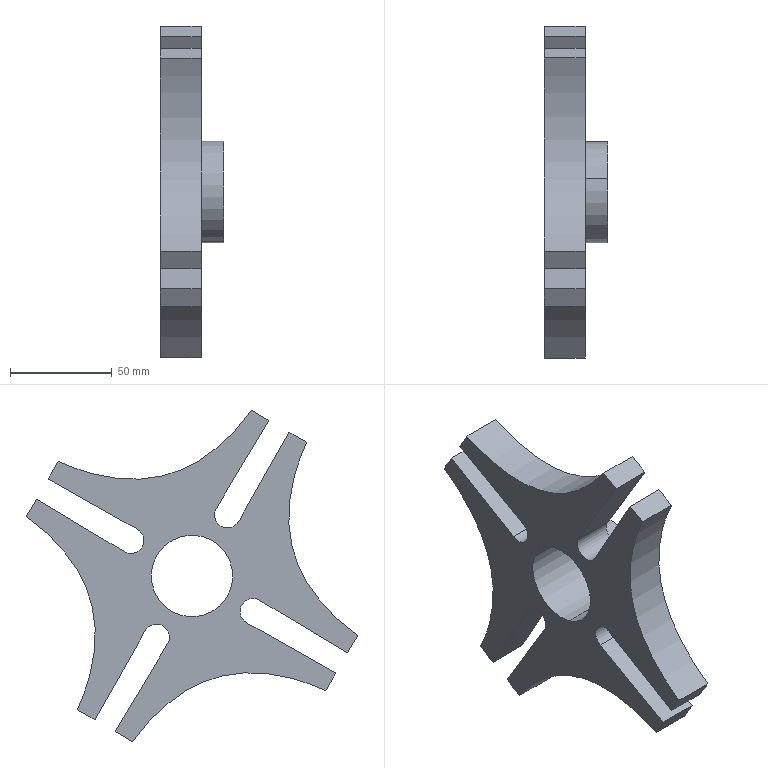Component | SolidWorks | GrooveWheel-2 | 1 solid | 33 faces | box 31 x 162.73 x 162.73 mm | volume 210042 mm3 | plane 19 | cylinder 10 | spline 4 | commonest cylinder face diameters 12.728 x6 40 x2 50 x2
STEP:
#1=CARTESIAN_POINT('',(15.611,0.8047,-8.688));
#2=VERTEX_POINT('',#1);
#3=CARTESIAN_POINT('',(15.611,0.4008,-10.21));
#4=VERTEX_POINT('',#3);
#5=CARTESIAN_POINT('',(15.611,0.6028,-9.449));
#6=DIRECTION('',(1.,0.,0.));
#7=DIRECTION('',(0.,-0.2564,-0.9666));
#8=AXIS2_PLACEMENT_3D('',#5,#6,#7);
#9=CIRCLE('',#8,0.7874);
#10=EDGE_CURVE('',#2,#4,#9,.T.);
#11=ORIENTED_EDGE('',*,*,#10,.T.);
#12=CARTESIAN_POINT('',(14.391,0.4008,-10.21));
#13=VERTEX_POINT('',#12);
#14=CARTESIAN_POINT('',(15.611,0.4008,-10.21));
#15=DIRECTION('',(-1.,0.,0.));
#16=VECTOR('',#15,39.37);
#17=LINE('',#14,#16);
#18=EDGE_CURVE('',#4,#13,#17,.T.);
#19=ORIENTED_EDGE('',*,*,#18,.T.);
#20=CARTESIAN_POINT('',(14.391,0.8047,-8.688));
#21=VERTEX_POINT('',#20);
#22=CARTESIAN_POINT('',(14.391,0.6028,-9.449));
#23=DIRECTION('',(1.,0.,0.));
#24=DIRECTION('',(0.,-0.2564,-0.9666));
#25=AXIS2_PLACEMENT_3D('',#22,#23,#24);
#26=CIRCLE('',#25,0.7874);
#27=EDGE_CURVE('',#21,#13,#26,.T.);
#28=ORIENTED_EDGE('',*,*,#27,.F.);
#29=CARTESIAN_POINT('',(15.611,0.8047,-8.688));
#30=DIRECTION('',(-1.,0.,0.));
#31=VECTOR('',#30,39.37);
#32=LINE('',#29,#31);
#33=EDGE_CURVE('',#2,#21,#32,.T.);
#34=ORIENTED_EDGE('',*,*,#33,.F.);
#35=EDGE_LOOP('',(#11,#19,#28,#34));
#36=FACE_OUTER_BOUND('',#35,.T.);
#37=CARTESIAN_POINT('',(15.611,0.6028,-9.449));
#38=DIRECTION('',(-1.,0.,0.));
#39=DIRECTION('',(0.,0.2564,0.9666));
#40=AXIS2_PLACEMENT_3D('',#37,#38,#39);
#41=CYLINDRICAL_SURFACE('',#40,0.7874);
#42=ADVANCED_FACE('',(#36),#41,.F.);
#43=CARTESIAN_POINT('',(15.611,0.3504,-10.4));
#44=VERTEX_POINT('',#43);
#45=CARTESIAN_POINT('',(15.611,0.8552,-8.497));
#46=VERTEX_POINT('',#45);
#47=CARTESIAN_POINT('',(15.611,0.6028,-9.449));
#48=DIRECTION('',(1.,0.,0.));
#49=DIRECTION('',(0.,-0.2564,-0.9666));
#50=AXIS2_PLACEMENT_3D('',#47,#48,#49);
#51=CIRCLE('',#50,0.9843);
#52=EDGE_CURVE('',#44,#46,#51,.T.);
#53=ORIENTED_EDGE('',*,*,#52,.F.);
#54=CARTESIAN_POINT('',(15.178,0.3504,-10.4));
#55=VERTEX_POINT('',#54);
#56=CARTESIAN_POINT('',(15.611,0.3504,-10.4));
#57=DIRECTION('',(-1.,0.,0.));
#58=VECTOR('',#57,39.37);
#59=LINE('',#56,#58);
#60=EDGE_CURVE('',#44,#55,#59,.T.);
#61=ORIENTED_EDGE('',*,*,#60,.T.);
#62=CARTESIAN_POINT('',(15.178,0.8552,-8.497));
#63=VERTEX_POINT('',#62);
#64=CARTESIAN_POINT('',(15.178,0.6028,-9.449));
#65=DIRECTION('',(1.,0.,0.));
#66=DIRECTION('',(0.,-0.2564,-0.9666));
#67=AXIS2_PLACEMENT_3D('',#64,#65,#66);
#68=CIRCLE('',#67,0.9843);
#69=EDGE_CURVE('',#55,#63,#68,.T.);
#70=ORIENTED_EDGE('',*,*,#69,.T.);
#71=CARTESIAN_POINT('',(15.611,0.8552,-8.497));
#72=DIRECTION('',(-1.,0.,0.));
#73=VECTOR('',#72,39.37);
#74=LINE('',#71,#73);
#75=EDGE_CURVE('',#46,#63,#74,.T.);
#76=ORIENTED_EDGE('',*,*,#75,.F.);
#77=EDGE_LOOP('',(#53,#61,#70,#76));
#78=FACE_OUTER_BOUND('',#77,.T.);
#79=CARTESIAN_POINT('',(15.611,0.6028,-9.449));
#80=DIRECTION('',(-1.,0.,0.));
#81=DIRECTION('',(0.,0.2564,0.9666));
#82=AXIS2_PLACEMENT_3D('',#79,#80,#81);
#83=CYLINDRICAL_SURFACE('',#82,0.9843);
#84=ADVANCED_FACE('',(#78),#83,.T.);
#85=CARTESIAN_POINT('',(15.178,1.508,-10.509));
#86=VERTEX_POINT('',#85);
#87=CARTESIAN_POINT('',(15.178,1.352,-10.386));
#88=VERTEX_POINT('',#87);
#89=CARTESIAN_POINT('',(15.178,1.288,-10.628));
#90=DIRECTION('',(1.,0.,0.));
#91=DIRECTION('',(0.,-0.2564,-0.9666));
#92=AXIS2_PLACEMENT_3D('',#89,#90,#91);
#93=CIRCLE('',#92,0.2505);
#94=EDGE_CURVE('',#86,#88,#93,.T.);
#95=ORIENTED_EDGE('',*,*,#94,.T.);
#96=CARTESIAN_POINT('',(14.391,1.352,-10.386));
#97=VERTEX_POINT('',#96);
#98=CARTESIAN_POINT('',(15.178,1.352,-10.386));
#99=DIRECTION('',(-1.,0.,0.));
#100=VECTOR('',#99,39.37);
#101=LINE('',#98,#100);
#102=EDGE_CURVE('',#88,#97,#101,.T.);
#103=ORIENTED_EDGE('',*,*,#102,.T.);
#104=CARTESIAN_POINT('',(14.391,1.508,-10.509));
#105=VERTEX_POINT('',#104);
#106=CARTESIAN_POINT('',(14.391,1.288,-10.628));
#107=DIRECTION('',(1.,0.,0.));
#108=DIRECTION('',(0.,-0.2564,-0.9666));
#109=AXIS2_PLACEMENT_3D('',#106,#107,#108);
#110=CIRCLE('',#109,0.2505);
#111=EDGE_CURVE('',#105,#97,#110,.T.);
#112=ORIENTED_EDGE('',*,*,#111,.F.);
#113=CARTESIAN_POINT('',(15.178,1.508,-10.509));
#114=DIRECTION('',(-1.,0.,0.));
#115=VECTOR('',#114,39.37);
#116=LINE('',#113,#115);
#117=EDGE_CURVE('',#86,#105,#116,.T.);
#118=ORIENTED_EDGE('',*,*,#117,.F.);
#119=EDGE_LOOP('',(#95,#103,#112,#118));
#120=FACE_OUTER_BOUND('',#119,.T.);
#121=CARTESIAN_POINT('',(15.178,1.288,-10.628));
#122=DIRECTION('',(-1.,0.,0.));
#123=DIRECTION('',(0.,0.2564,0.9666));
#124=AXIS2_PLACEMENT_3D('',#121,#122,#123);
#125=CYLINDRICAL_SURFACE('',#124,0.2505);
#126=ADVANCED_FACE('',(#120),#125,.F.);
#127=CARTESIAN_POINT('',(15.178,-0.4572,-10.354));
#128=VERTEX_POINT('',#127);
#129=CARTESIAN_POINT('',(15.178,-0.5127,-9.892));
#130=VERTEX_POINT('',#129);
#131=CARTESIAN_POINT('',(15.178,-0.5769,-10.134));
#132=DIRECTION('',(1.,0.,0.));
#133=DIRECTION('',(0.,-0.2564,-0.9666));
#134=AXIS2_PLACEMENT_3D('',#131,#132,#133);
#135=CIRCLE('',#134,0.2505);
#136=EDGE_CURVE('',#128,#130,#135,.T.);
#137=ORIENTED_EDGE('',*,*,#136,.T.);
#138=CARTESIAN_POINT('',(14.391,-0.5127,-9.892));
#139=VERTEX_POINT('',#138);
#140=CARTESIAN_POINT('',(15.178,-0.5127,-9.892));
#141=DIRECTION('',(-1.,0.,0.));
#142=VECTOR('',#141,39.37);
#143=LINE('',#140,#142);
#144=EDGE_CURVE('',#130,#139,#143,.T.);
#145=ORIENTED_EDGE('',*,*,#144,.T.);
#146=CARTESIAN_POINT('',(14.391,-0.4572,-10.354));
#147=VERTEX_POINT('',#146);
#148=CARTESIAN_POINT('',(14.391,-0.5769,-10.134));
#149=DIRECTION('',(1.,0.,0.));
#150=DIRECTION('',(0.,-0.2564,-0.9666));
#151=AXIS2_PLACEMENT_3D('',#148,#149,#150);
#152=CIRCLE('',#151,0.2505);
#153=EDGE_CURVE('',#147,#139,#152,.T.);
#154=ORIENTED_EDGE('',*,*,#153,.F.);
#155=CARTESIAN_POINT('',(15.178,-0.4572,-10.354));
#156=DIRECTION('',(-1.,0.,0.));
#157=VECTOR('',#156,39.37);
#158=LINE('',#155,#157);
#159=EDGE_CURVE('',#128,#147,#158,.T.);
#160=ORIENTED_EDGE('',*,*,#159,.F.);
#161=EDGE_LOOP('',(#137,#145,#154,#160));
#162=FACE_OUTER_BOUND('',#161,.T.);
#163=CARTESIAN_POINT('',(15.178,-0.5769,-10.134));
#164=DIRECTION('',(-1.,0.,0.));
#165=DIRECTION('',(0.,0.2564,0.9666));
#166=AXIS2_PLACEMENT_3D('',#163,#164,#165);
#167=CYLINDRICAL_SURFACE('',#166,0.2505);
#168=ADVANCED_FACE('',(#162),#167,.F.);
#169=CARTESIAN_POINT('',(15.178,-0.5444,-6.246));
#170=VERTEX_POINT('',#169);
#171=CARTESIAN_POINT('',(15.178,3.187,-7.236));
#172=VERTEX_POINT('',#171);
#173=CARTESIAN_POINT('',(15.178,-0.5444,-6.246));
#174=CARTESIAN_POINT('',(15.178,0.9175,-8.263));
#175=CARTESIAN_POINT('',(15.178,3.187,-7.236));
#176=B_SPLINE_CURVE_WITH_KNOTS('',2,(#173,#174,#175),.UNSPECIFIED.,.F.,.F.,(3,3),(0.,1.),.UNSPECIFIED.);
#177=EDGE_CURVE('',#170,#172,#176,.T.);
#178=ORIENTED_EDGE('',*,*,#177,.F.);
#179=CARTESIAN_POINT('',(15.178,-0.8821,-6.448));
#180=VERTEX_POINT('',#179);
#181=CARTESIAN_POINT('',(15.178,-1.113,-6.587));
#182=DIRECTION('',(0.,0.8576,0.5143));
#183=VECTOR('',#182,39.37);
#184=LINE('',#181,#183);
#185=EDGE_CURVE('',#180,#170,#184,.T.);
#186=ORIENTED_EDGE('',*,*,#185,.F.);
#187=CARTESIAN_POINT('',(15.178,0.1309,-8.137));
#188=VERTEX_POINT('',#187);
#189=CARTESIAN_POINT('',(15.178,0.8341,-9.31));
#190=DIRECTION('',(0.,0.5143,-0.8576));
#191=VECTOR('',#190,39.37);
#192=LINE('',#189,#191);
#193=EDGE_CURVE('',#180,#188,#192,.T.);
#194=ORIENTED_EDGE('',*,*,#193,.T.);
#195=CARTESIAN_POINT('',(15.178,-0.3023,-8.389));
#196=VERTEX_POINT('',#195);
#197=CARTESIAN_POINT('',(15.178,-0.08218,-8.269));
#198=DIRECTION('',(1.,0.,0.));
#199=DIRECTION('',(0.,-0.2564,-0.9666));
#200=AXIS2_PLACEMENT_3D('',#197,#198,#199);
#201=CIRCLE('',#200,0.2505);
#202=EDGE_CURVE('',#196,#188,#201,.T.);
#203=ORIENTED_EDGE('',*,*,#202,.F.);
#204=CARTESIAN_POINT('',(15.178,-1.267,-6.672));
#205=VERTEX_POINT('',#204);
#206=CARTESIAN_POINT('',(15.178,0.3676,-9.581));
#207=DIRECTION('',(0.,0.4899,-0.8718));
#208=VECTOR('',#207,39.37);
#209=LINE('',#206,#208);
#210=EDGE_CURVE('',#205,#196,#209,.T.);
#211=ORIENTED_EDGE('',*,*,#210,.F.);
#212=CARTESIAN_POINT('',(15.178,-1.61,-6.865));
#213=VERTEX_POINT('',#212);
#214=CARTESIAN_POINT('',(15.178,-1.032,-6.54));
#215=DIRECTION('',(0.,-0.8718,-0.4899));
#216=VECTOR('',#215,39.37);
#217=LINE('',#214,#216);
#218=EDGE_CURVE('',#205,#213,#217,.T.);
#219=ORIENTED_EDGE('',*,*,#218,.T.);
#220=CARTESIAN_POINT('',(15.178,-2.601,-10.596));
#221=VERTEX_POINT('',#220);
#222=CARTESIAN_POINT('',(15.178,-2.601,-10.596));
#223=CARTESIAN_POINT('',(15.178,-0.5834,-9.134));
#224=CARTESIAN_POINT('',(15.178,-1.61,-6.865));
#225=B_SPLINE_CURVE_WITH_KNOTS('',2,(#222,#223,#224),.UNSPECIFIED.,.F.,.F.,(3,3),(0.,1.),.UNSPECIFIED.);
#226=EDGE_CURVE('',#221,#213,#225,.T.);
#227=ORIENTED_EDGE('',*,*,#226,.F.);
#228=CARTESIAN_POINT('',(15.178,-2.398,-10.934));
#229=VERTEX_POINT('',#228);
#230=CARTESIAN_POINT('',(15.178,-2.259,-11.165));
#231=DIRECTION('',(0.,-0.5143,0.8576));
#232=VECTOR('',#231,39.37);
#233=LINE('',#230,#232);
#234=EDGE_CURVE('',#229,#221,#233,.T.);
#235=ORIENTED_EDGE('',*,*,#234,.F.);
#236=CARTESIAN_POINT('',(15.178,-0.7088,-9.921));
#237=VERTEX_POINT('',#236);
#238=CARTESIAN_POINT('',(15.178,0.4641,-9.217));
#239=DIRECTION('',(0.,0.8576,0.5143));
#240=VECTOR('',#239,39.37);
#241=LINE('',#238,#240);
#242=EDGE_CURVE('',#229,#237,#241,.T.);
#243=ORIENTED_EDGE('',*,*,#242,.T.);
#244=CARTESIAN_POINT('',(15.178,-0.5769,-10.134));
#245=DIRECTION('',(1.,0.,0.));
#246=DIRECTION('',(0.,-0.2564,-0.9666));
#247=AXIS2_PLACEMENT_3D('',#244,#245,#246);
#248=CIRCLE('',#247,0.2505);
#249=EDGE_CURVE('',#130,#237,#248,.T.);
#250=ORIENTED_EDGE('',*,*,#249,.F.);
#251=ORIENTED_EDGE('',*,*,#136,.F.);
#252=CARTESIAN_POINT('',(15.178,-2.174,-11.319));
#253=VERTEX_POINT('',#252);
#254=CARTESIAN_POINT('',(15.178,0.7349,-9.684));
#255=DIRECTION('',(0.,0.8718,0.4899));
#256=VECTOR('',#255,39.37);
#257=LINE('',#254,#256);
#258=EDGE_CURVE('',#253,#128,#257,.T.);
#259=ORIENTED_EDGE('',*,*,#258,.F.);
#260=CARTESIAN_POINT('',(15.178,-1.982,-11.662));
#261=VERTEX_POINT('',#260);
#262=CARTESIAN_POINT('',(15.178,-2.307,-11.084));
#263=DIRECTION('',(0.,0.4899,-0.8718));
#264=VECTOR('',#263,39.37);
#265=LINE('',#262,#264);
#266=EDGE_CURVE('',#253,#261,#265,.T.);
#267=ORIENTED_EDGE('',*,*,#266,.T.);
#268=CARTESIAN_POINT('',(15.178,1.75,-12.652));
#269=VERTEX_POINT('',#268);
#270=CARTESIAN_POINT('',(15.178,1.75,-12.652));
#271=CARTESIAN_POINT('',(15.178,0.2881,-10.635));
#272=CARTESIAN_POINT('',(15.178,-1.982,-11.662));
#273=B_SPLINE_CURVE_WITH_KNOTS('',2,(#270,#271,#272),.UNSPECIFIED.,.F.,.F.,(3,3),(0.,1.),.UNSPECIFIED.);
#274=EDGE_CURVE('',#269,#261,#273,.T.);
#275=ORIENTED_EDGE('',*,*,#274,.F.);
#276=CARTESIAN_POINT('',(15.178,2.088,-12.45));
#277=VERTEX_POINT('',#276);
#278=CARTESIAN_POINT('',(15.178,2.319,-12.311));
#279=DIRECTION('',(0.,-0.8576,-0.5143));
#280=VECTOR('',#279,39.37);
#281=LINE('',#278,#280);
#282=EDGE_CURVE('',#277,#269,#281,.T.);
#283=ORIENTED_EDGE('',*,*,#282,.F.);
#284=CARTESIAN_POINT('',(15.178,1.075,-10.76));
#285=VERTEX_POINT('',#284);
#286=CARTESIAN_POINT('',(15.178,0.3714,-9.588));
#287=DIRECTION('',(0.,-0.5143,0.8576));
#288=VECTOR('',#287,39.37);
#289=LINE('',#286,#288);
#290=EDGE_CURVE('',#277,#285,#289,.T.);
#291=ORIENTED_EDGE('',*,*,#290,.T.);
#292=CARTESIAN_POINT('',(15.178,1.288,-10.628));
#293=DIRECTION('',(1.,0.,0.));
#294=DIRECTION('',(0.,-0.2564,-0.9666));
#295=AXIS2_PLACEMENT_3D('',#292,#293,#294);
#296=CIRCLE('',#295,0.2505);
#297=EDGE_CURVE('',#88,#285,#296,.T.);
#298=ORIENTED_EDGE('',*,*,#297,.F.);
#299=ORIENTED_EDGE('',*,*,#94,.F.);
#300=CARTESIAN_POINT('',(15.178,2.473,-12.226));
#301=VERTEX_POINT('',#300);
#302=CARTESIAN_POINT('',(15.178,0.8379,-9.317));
#303=DIRECTION('',(0.,-0.4899,0.8718));
#304=VECTOR('',#303,39.37);
#305=LINE('',#302,#304);
#306=EDGE_CURVE('',#301,#86,#305,.T.);
#307=ORIENTED_EDGE('',*,*,#306,.F.);
#308=CARTESIAN_POINT('',(15.178,2.816,-12.033));
#309=VERTEX_POINT('',#308);
#310=CARTESIAN_POINT('',(15.178,2.238,-12.358));
#311=DIRECTION('',(0.,0.8718,0.4899));
#312=VECTOR('',#311,39.37);
#313=LINE('',#310,#312);
#314=EDGE_CURVE('',#301,#309,#313,.T.);
#315=ORIENTED_EDGE('',*,*,#314,.T.);
#316=CARTESIAN_POINT('',(15.178,3.806,-8.302));
#317=VERTEX_POINT('',#316);
#318=CARTESIAN_POINT('',(15.178,3.806,-8.302));
#319=CARTESIAN_POINT('',(15.178,1.789,-9.764));
#320=CARTESIAN_POINT('',(15.178,2.816,-12.033));
#321=B_SPLINE_CURVE_WITH_KNOTS('',2,(#318,#319,#320),.UNSPECIFIED.,.F.,.F.,(3,3),(0.,1.),.UNSPECIFIED.);
#322=EDGE_CURVE('',#317,#309,#321,.T.);
#323=ORIENTED_EDGE('',*,*,#322,.F.);
#324=CARTESIAN_POINT('',(15.178,3.604,-7.964));
#325=VERTEX_POINT('',#324);
#326=CARTESIAN_POINT('',(15.178,3.465,-7.733));
#327=DIRECTION('',(0.,0.5143,-0.8576));
#328=VECTOR('',#327,39.37);
#329=LINE('',#326,#328);
#330=EDGE_CURVE('',#325,#317,#329,.T.);
#331=ORIENTED_EDGE('',*,*,#330,.F.);
#332=CARTESIAN_POINT('',(15.178,1.914,-8.977));
#333=VERTEX_POINT('',#332);
#334=CARTESIAN_POINT('',(15.178,0.7415,-9.68));
#335=DIRECTION('',(0.,-0.8576,-0.5143));
#336=VECTOR('',#335,39.37);
#337=LINE('',#334,#336);
#338=EDGE_CURVE('',#325,#333,#337,.T.);
#339=ORIENTED_EDGE('',*,*,#338,.T.);
#340=CARTESIAN_POINT('',(15.178,1.663,-8.544));
#341=VERTEX_POINT('',#340);
#342=CARTESIAN_POINT('',(15.178,1.782,-8.764));
#343=DIRECTION('',(1.,0.,0.));
#344=DIRECTION('',(0.,-0.2564,-0.9666));
#345=AXIS2_PLACEMENT_3D('',#342,#343,#344);
#346=CIRCLE('',#345,0.2505);
#347=EDGE_CURVE('',#341,#333,#346,.T.);
#348=ORIENTED_EDGE('',*,*,#347,.F.);
#349=CARTESIAN_POINT('',(15.178,3.38,-7.579));
#350=VERTEX_POINT('',#349);
#351=CARTESIAN_POINT('',(15.178,0.4706,-9.214));
#352=DIRECTION('',(0.,-0.8718,-0.4899));
#353=VECTOR('',#352,39.37);
#354=LINE('',#351,#353);
#355=EDGE_CURVE('',#350,#341,#354,.T.);
#356=ORIENTED_EDGE('',*,*,#355,.F.);
#357=CARTESIAN_POINT('',(15.178,3.512,-7.814));
#358=DIRECTION('',(0.,-0.4899,0.8718));
#359=VECTOR('',#358,39.37);
#360=LINE('',#357,#359);
#361=EDGE_CURVE('',#350,#172,#360,.T.);
#362=ORIENTED_EDGE('',*,*,#361,.T.);
#363=EDGE_LOOP('',(#178,#186,#194,#203,#211,#219,#227,#235,#243,#250,#251,#259,#267,#275,#283,#291,#298,#299,#307,#315,#323,#331,#339,#348,#356,#362));
#364=FACE_OUTER_BOUND('',#363,.T.);
#365=CARTESIAN_POINT('',(15.178,0.6028,-9.449));
#366=DIRECTION('',(1.,0.,0.));
#367=DIRECTION('',(0.,-0.2564,-0.9666));
#368=AXIS2_PLACEMENT_3D('',#365,#366,#367);
#369=CIRCLE('',#368,0.9843);
#370=EDGE_CURVE('',#63,#55,#369,.T.);
#371=ORIENTED_EDGE('',*,*,#370,.F.);
#372=ORIENTED_EDGE('',*,*,#69,.F.);
#373=EDGE_LOOP('',(#371,#372));
#374=FACE_BOUND('',#373,.T.);
#375=CARTESIAN_POINT('',(15.178,0.6028,-9.449));
#376=DIRECTION('',(1.,0.,0.));
#377=DIRECTION('',(0.,-0.2564,-0.9666));
#378=AXIS2_PLACEMENT_3D('',#375,#376,#377);
#379=PLANE('',#378);
#380=ADVANCED_FACE('',(#364,#374),#379,.T.);
#381=CARTESIAN_POINT('',(14.391,-0.5444,-6.246));
#382=VERTEX_POINT('',#381);
#383=CARTESIAN_POINT('',(14.391,3.187,-7.236));
#384=VERTEX_POINT('',#383);
#385=CARTESIAN_POINT('',(14.391,-0.5444,-6.246));
#386=CARTESIAN_POINT('',(14.391,0.9175,-8.263));
#387=CARTESIAN_POINT('',(14.391,3.187,-7.236));
#388=B_SPLINE_CURVE_WITH_KNOTS('',2,(#385,#386,#387),.UNSPECIFIED.,.F.,.F.,(3,3),(0.,1.),.UNSPECIFIED.);
#389=EDGE_CURVE('',#382,#384,#388,.T.);
#390=ORIENTED_EDGE('',*,*,#389,.F.);
#391=CARTESIAN_POINT('',(15.178,-0.5444,-6.246));
#392=DIRECTION('',(-1.,0.,0.));
#393=VECTOR('',#392,39.37);
#394=LINE('',#391,#393);
#395=EDGE_CURVE('',#170,#382,#394,.T.);
#396=ORIENTED_EDGE('',*,*,#395,.F.);
#397=ORIENTED_EDGE('',*,*,#177,.T.);
#398=CARTESIAN_POINT('',(15.178,3.187,-7.236));
#399=DIRECTION('',(-1.,0.,0.));
#400=VECTOR('',#399,39.37);
#401=LINE('',#398,#400);
#402=EDGE_CURVE('',#172,#384,#401,.T.);
#403=ORIENTED_EDGE('',*,*,#402,.T.);
#404=EDGE_LOOP('',(#390,#396,#397,#403));
#405=FACE_OUTER_BOUND('',#404,.T.);
#406=CARTESIAN_POINT('',(15.178,-0.5444,-6.246));
#407=CARTESIAN_POINT('',(14.391,-0.5444,-6.246));
#408=CARTESIAN_POINT('',(15.178,0.9175,-8.263));
#409=CARTESIAN_POINT('',(14.391,0.9175,-8.263));
#410=CARTESIAN_POINT('',(15.178,3.187,-7.236));
#411=CARTESIAN_POINT('',(14.391,3.187,-7.236));
#412=B_SPLINE_SURFACE_WITH_KNOTS('',2,1,((#406,#407),(#408,#409),(#410,#411)),.UNSPECIFIED.,.F.,.F.,.F.,(3,3),(2,2),(0.,1.),(0.,1.),.UNSPECIFIED.);
#413=ADVANCED_FACE('',(#405),#412,.T.);
#414=CARTESIAN_POINT('',(14.391,-0.8821,-6.448));
#415=VERTEX_POINT('',#414);
#416=CARTESIAN_POINT('',(14.391,-1.113,-6.587));
#417=DIRECTION('',(0.,0.8576,0.5143));
#418=VECTOR('',#417,39.37);
#419=LINE('',#416,#418);
#420=EDGE_CURVE('',#415,#382,#419,.T.);
#421=ORIENTED_EDGE('',*,*,#420,.F.);
#422=CARTESIAN_POINT('',(15.178,-0.8821,-6.448));
#423=DIRECTION('',(-1.,0.,0.));
#424=VECTOR('',#423,39.37);
#425=LINE('',#422,#424);
#426=EDGE_CURVE('',#180,#415,#425,.T.);
#427=ORIENTED_EDGE('',*,*,#426,.F.);
#428=ORIENTED_EDGE('',*,*,#185,.T.);
#429=ORIENTED_EDGE('',*,*,#395,.T.);
#430=EDGE_LOOP('',(#421,#427,#428,#429));
#431=FACE_OUTER_BOUND('',#430,.T.);
#432=CARTESIAN_POINT('',(15.178,-1.113,-6.587));
#433=DIRECTION('',(0.,-0.5143,0.8576));
#434=DIRECTION('',(0.,-0.8576,-0.5143));
#435=AXIS2_PLACEMENT_3D('',#432,#433,#434);
#436=PLANE('',#435);
#437=ADVANCED_FACE('',(#431),#436,.T.);
#438=CARTESIAN_POINT('',(14.391,0.1309,-8.137));
#439=VERTEX_POINT('',#438);
#440=CARTESIAN_POINT('',(14.391,0.8341,-9.31));
#441=DIRECTION('',(0.,0.5143,-0.8576));
#442=VECTOR('',#441,39.37);
#443=LINE('',#440,#442);
#444=EDGE_CURVE('',#415,#439,#443,.T.);
#445=ORIENTED_EDGE('',*,*,#444,.T.);
#446=CARTESIAN_POINT('',(15.178,0.1309,-8.137));
#447=DIRECTION('',(-1.,0.,0.));
#448=VECTOR('',#447,39.37);
#449=LINE('',#446,#448);
#450=EDGE_CURVE('',#188,#439,#449,.T.);
#451=ORIENTED_EDGE('',*,*,#450,.F.);
#452=ORIENTED_EDGE('',*,*,#193,.F.);
#453=ORIENTED_EDGE('',*,*,#426,.T.);
#454=EDGE_LOOP('',(#445,#451,#452,#453));
#455=FACE_OUTER_BOUND('',#454,.T.);
#456=CARTESIAN_POINT('',(15.178,0.8341,-9.31));
#457=DIRECTION('',(0.,0.8576,0.5143));
#458=DIRECTION('',(0.,-0.5143,0.8576));
#459=AXIS2_PLACEMENT_3D('',#456,#457,#458);
#460=PLANE('',#459);
#461=ADVANCED_FACE('',(#455),#460,.F.);
#462=CARTESIAN_POINT('',(14.391,-0.3023,-8.389));
#463=VERTEX_POINT('',#462);
#464=CARTESIAN_POINT('',(14.391,-0.08218,-8.269));
#465=DIRECTION('',(1.,0.,0.));
#466=DIRECTION('',(0.,-0.2564,-0.9666));
#467=AXIS2_PLACEMENT_3D('',#464,#465,#466);
#468=CIRCLE('',#467,0.2505);
#469=EDGE_CURVE('',#463,#439,#468,.T.);
#470=ORIENTED_EDGE('',*,*,#469,.F.);
#471=CARTESIAN_POINT('',(15.178,-0.3023,-8.389));
#472=DIRECTION('',(-1.,0.,0.));
#473=VECTOR('',#472,39.37);
#474=LINE('',#471,#473);
#475=EDGE_CURVE('',#196,#463,#474,.T.);
#476=ORIENTED_EDGE('',*,*,#475,.F.);
#477=ORIENTED_EDGE('',*,*,#202,.T.);
#478=ORIENTED_EDGE('',*,*,#450,.T.);
#479=EDGE_LOOP('',(#470,#476,#477,#478));
#480=FACE_OUTER_BOUND('',#479,.T.);
#481=CARTESIAN_POINT('',(15.178,-0.08218,-8.269));
#482=DIRECTION('',(-1.,0.,0.));
#483=DIRECTION('',(0.,0.2564,0.9666));
#484=AXIS2_PLACEMENT_3D('',#481,#482,#483);
#485=CYLINDRICAL_SURFACE('',#484,0.2505);
#486=ADVANCED_FACE('',(#480),#485,.F.);
#487=CARTESIAN_POINT('',(14.391,-1.267,-6.672));
#488=VERTEX_POINT('',#487);
#489=CARTESIAN_POINT('',(14.391,0.3676,-9.581));
#490=DIRECTION('',(0.,0.4899,-0.8718));
#491=VECTOR('',#490,39.37);
#492=LINE('',#489,#491);
#493=EDGE_CURVE('',#488,#463,#492,.T.);
#494=ORIENTED_EDGE('',*,*,#493,.F.);
#495=CARTESIAN_POINT('',(15.178,-1.267,-6.672));
#496=DIRECTION('',(-1.,0.,0.));
#497=VECTOR('',#496,39.37);
#498=LINE('',#495,#497);
#499=EDGE_CURVE('',#205,#488,#498,.T.);
#500=ORIENTED_EDGE('',*,*,#499,.F.);
#501=ORIENTED_EDGE('',*,*,#210,.T.);
#502=ORIENTED_EDGE('',*,*,#475,.T.);
#503=EDGE_LOOP('',(#494,#500,#501,#502));
#504=FACE_OUTER_BOUND('',#503,.T.);
#505=CARTESIAN_POINT('',(15.178,0.3676,-9.581));
#506=DIRECTION('',(0.,0.8718,0.4899));
#507=DIRECTION('',(0.,-0.4899,0.8718));
#508=AXIS2_PLACEMENT_3D('',#505,#506,#507);
#509=PLANE('',#508);
#510=ADVANCED_FACE('',(#504),#509,.T.);
#511=CARTESIAN_POINT('',(14.391,-1.61,-6.865));
#512=VERTEX_POINT('',#511);
#513=CARTESIAN_POINT('',(14.391,-1.032,-6.54));
#514=DIRECTION('',(0.,-0.8718,-0.4899));
#515=VECTOR('',#514,39.37);
#516=LINE('',#513,#515);
#517=EDGE_CURVE('',#488,#512,#516,.T.);
#518=ORIENTED_EDGE('',*,*,#517,.T.);
#519=CARTESIAN_POINT('',(15.178,-1.61,-6.865));
#520=DIRECTION('',(-1.,0.,0.));
#521=VECTOR('',#520,39.37);
#522=LINE('',#519,#521);
#523=EDGE_CURVE('',#213,#512,#522,.T.);
#524=ORIENTED_EDGE('',*,*,#523,.F.);
#525=ORIENTED_EDGE('',*,*,#218,.F.);
#526=ORIENTED_EDGE('',*,*,#499,.T.);
#527=EDGE_LOOP('',(#518,#524,#525,#526));
#528=FACE_OUTER_BOUND('',#527,.T.);
#529=CARTESIAN_POINT('',(15.178,-1.032,-6.54));
#530=DIRECTION('',(0.,0.4899,-0.8718));
#531=DIRECTION('',(0.,0.8718,0.4899));
#532=AXIS2_PLACEMENT_3D('',#529,#530,#531);
#533=PLANE('',#532);
#534=ADVANCED_FACE('',(#528),#533,.F.);
#535=CARTESIAN_POINT('',(14.391,-2.601,-10.596));
#536=VERTEX_POINT('',#535);
#537=CARTESIAN_POINT('',(14.391,-2.601,-10.596));
#538=CARTESIAN_POINT('',(14.391,-0.5834,-9.134));
#539=CARTESIAN_POINT('',(14.391,-1.61,-6.865));
#540=B_SPLINE_CURVE_WITH_KNOTS('',2,(#537,#538,#539),.UNSPECIFIED.,.F.,.F.,(3,3),(0.,1.),.UNSPECIFIED.);
#541=EDGE_CURVE('',#536,#512,#540,.T.);
#542=ORIENTED_EDGE('',*,*,#541,.F.);
#543=CARTESIAN_POINT('',(15.178,-2.601,-10.596));
#544=DIRECTION('',(-1.,0.,0.));
#545=VECTOR('',#544,39.37);
#546=LINE('',#543,#545);
#547=EDGE_CURVE('',#221,#536,#546,.T.);
#548=ORIENTED_EDGE('',*,*,#547,.F.);
#549=ORIENTED_EDGE('',*,*,#226,.T.);
#550=ORIENTED_EDGE('',*,*,#523,.T.);
#551=EDGE_LOOP('',(#542,#548,#549,#550));
#552=FACE_OUTER_BOUND('',#551,.T.);
#553=CARTESIAN_POINT('',(15.178,-2.601,-10.596));
#554=CARTESIAN_POINT('',(14.391,-2.601,-10.596));
#555=CARTESIAN_POINT('',(15.178,-0.5834,-9.134));
#556=CARTESIAN_POINT('',(14.391,-0.5834,-9.134));
#557=CARTESIAN_POINT('',(15.178,-1.61,-6.865));
#558=CARTESIAN_POINT('',(14.391,-1.61,-6.865));
#559=B_SPLINE_SURFACE_WITH_KNOTS('',2,1,((#553,#554),(#555,#556),(#557,#558)),.UNSPECIFIED.,.F.,.F.,.F.,(3,3),(2,2),(0.,1.),(0.,1.),.UNSPECIFIED.);
#560=ADVANCED_FACE('',(#552),#559,.T.);
#561=CARTESIAN_POINT('',(14.391,-2.398,-10.934));
#562=VERTEX_POINT('',#561);
#563=CARTESIAN_POINT('',(14.391,-2.259,-11.165));
#564=DIRECTION('',(0.,-0.5143,0.8576));
#565=VECTOR('',#564,39.37);
#566=LINE('',#563,#565);
#567=EDGE_CURVE('',#562,#536,#566,.T.);
#568=ORIENTED_EDGE('',*,*,#567,.F.);
#569=CARTESIAN_POINT('',(15.178,-2.398,-10.934));
#570=DIRECTION('',(-1.,0.,0.));
#571=VECTOR('',#570,39.37);
#572=LINE('',#569,#571);
#573=EDGE_CURVE('',#229,#562,#572,.T.);
#574=ORIENTED_EDGE('',*,*,#573,.F.);
#575=ORIENTED_EDGE('',*,*,#234,.T.);
#576=ORIENTED_EDGE('',*,*,#547,.T.);
#577=EDGE_LOOP('',(#568,#574,#575,#576));
#578=FACE_OUTER_BOUND('',#577,.T.);
#579=CARTESIAN_POINT('',(15.178,-2.259,-11.165));
#580=DIRECTION('',(0.,-0.8576,-0.5143));
#581=DIRECTION('',(0.,0.5143,-0.8576));
#582=AXIS2_PLACEMENT_3D('',#579,#580,#581);
#583=PLANE('',#582);
#584=ADVANCED_FACE('',(#578),#583,.T.);
#585=CARTESIAN_POINT('',(14.391,-0.7088,-9.921));
#586=VERTEX_POINT('',#585);
#587=CARTESIAN_POINT('',(14.391,0.4641,-9.217));
#588=DIRECTION('',(0.,0.8576,0.5143));
#589=VECTOR('',#588,39.37);
#590=LINE('',#587,#589);
#591=EDGE_CURVE('',#562,#586,#590,.T.);
#592=ORIENTED_EDGE('',*,*,#591,.T.);
#593=CARTESIAN_POINT('',(15.178,-0.7088,-9.921));
#594=DIRECTION('',(-1.,0.,0.));
#595=VECTOR('',#594,39.37);
#596=LINE('',#593,#595);
#597=EDGE_CURVE('',#237,#586,#596,.T.);
#598=ORIENTED_EDGE('',*,*,#597,.F.);
#599=ORIENTED_EDGE('',*,*,#242,.F.);
#600=ORIENTED_EDGE('',*,*,#573,.T.);
#601=EDGE_LOOP('',(#592,#598,#599,#600));
#602=FACE_OUTER_BOUND('',#601,.T.);
#603=CARTESIAN_POINT('',(15.178,0.4641,-9.217));
#604=DIRECTION('',(0.,-0.5143,0.8576));
#605=DIRECTION('',(0.,-0.8576,-0.5143));
#606=AXIS2_PLACEMENT_3D('',#603,#604,#605);
#607=PLANE('',#606);
#608=ADVANCED_FACE('',(#602),#607,.F.);
#609=ORIENTED_EDGE('',*,*,#144,.F.);
#610=ORIENTED_EDGE('',*,*,#249,.T.);
#611=ORIENTED_EDGE('',*,*,#597,.T.);
#612=CARTESIAN_POINT('',(14.391,-0.5769,-10.134));
#613=DIRECTION('',(1.,0.,0.));
#614=DIRECTION('',(0.,-0.2564,-0.9666));
#615=AXIS2_PLACEMENT_3D('',#612,#613,#614);
#616=CIRCLE('',#615,0.2505);
#617=EDGE_CURVE('',#139,#586,#616,.T.);
#618=ORIENTED_EDGE('',*,*,#617,.F.);
#619=EDGE_LOOP('',(#609,#610,#611,#618));
#620=FACE_OUTER_BOUND('',#619,.T.);
#621=CARTESIAN_POINT('',(15.178,-0.5769,-10.134));
#622=DIRECTION('',(-1.,0.,0.));
#623=DIRECTION('',(0.,0.2564,0.9666));
#624=AXIS2_PLACEMENT_3D('',#621,#622,#623);
#625=CYLINDRICAL_SURFACE('',#624,0.2505);
#626=ADVANCED_FACE('',(#620),#625,.F.);
#627=CARTESIAN_POINT('',(14.391,-2.174,-11.319));
#628=VERTEX_POINT('',#627);
#629=CARTESIAN_POINT('',(14.391,0.7349,-9.684));
#630=DIRECTION('',(0.,0.8718,0.4899));
#631=VECTOR('',#630,39.37);
#632=LINE('',#629,#631);
#633=EDGE_CURVE('',#628,#147,#632,.T.);
#634=ORIENTED_EDGE('',*,*,#633,.F.);
#635=CARTESIAN_POINT('',(15.178,-2.174,-11.319));
#636=DIRECTION('',(-1.,0.,0.));
#637=VECTOR('',#636,39.37);
#638=LINE('',#635,#637);
#639=EDGE_CURVE('',#253,#628,#638,.T.);
#640=ORIENTED_EDGE('',*,*,#639,.F.);
#641=ORIENTED_EDGE('',*,*,#258,.T.);
#642=ORIENTED_EDGE('',*,*,#159,.T.);
#643=EDGE_LOOP('',(#634,#640,#641,#642));
#644=FACE_OUTER_BOUND('',#643,.T.);
#645=CARTESIAN_POINT('',(15.178,0.7349,-9.684));
#646=DIRECTION('',(0.,-0.4899,0.8718));
#647=DIRECTION('',(0.,-0.8718,-0.4899));
#648=AXIS2_PLACEMENT_3D('',#645,#646,#647);
#649=PLANE('',#648);
#650=ADVANCED_FACE('',(#644),#649,.T.);
#651=CARTESIAN_POINT('',(14.391,-1.982,-11.662));
#652=VERTEX_POINT('',#651);
#653=CARTESIAN_POINT('',(14.391,-2.307,-11.084));
#654=DIRECTION('',(0.,0.4899,-0.8718));
#655=VECTOR('',#654,39.37);
#656=LINE('',#653,#655);
#657=EDGE_CURVE('',#628,#652,#656,.T.);
#658=ORIENTED_EDGE('',*,*,#657,.T.);
#659=CARTESIAN_POINT('',(15.178,-1.982,-11.662));
#660=DIRECTION('',(-1.,0.,0.));
#661=VECTOR('',#660,39.37);
#662=LINE('',#659,#661);
#663=EDGE_CURVE('',#261,#652,#662,.T.);
#664=ORIENTED_EDGE('',*,*,#663,.F.);
#665=ORIENTED_EDGE('',*,*,#266,.F.);
#666=ORIENTED_EDGE('',*,*,#639,.T.);
#667=EDGE_LOOP('',(#658,#664,#665,#666));
#668=FACE_OUTER_BOUND('',#667,.T.);
#669=CARTESIAN_POINT('',(15.178,-2.307,-11.084));
#670=DIRECTION('',(0.,0.8718,0.4899));
#671=DIRECTION('',(0.,-0.4899,0.8718));
#672=AXIS2_PLACEMENT_3D('',#669,#670,#671);
#673=PLANE('',#672);
#674=ADVANCED_FACE('',(#668),#673,.F.);
#675=CARTESIAN_POINT('',(14.391,1.75,-12.652));
#676=VERTEX_POINT('',#675);
#677=CARTESIAN_POINT('',(14.391,1.75,-12.652));
#678=CARTESIAN_POINT('',(14.391,0.2881,-10.635));
#679=CARTESIAN_POINT('',(14.391,-1.982,-11.662));
#680=B_SPLINE_CURVE_WITH_KNOTS('',2,(#677,#678,#679),.UNSPECIFIED.,.F.,.F.,(3,3),(0.,1.),.UNSPECIFIED.);
#681=EDGE_CURVE('',#676,#652,#680,.T.);
#682=ORIENTED_EDGE('',*,*,#681,.F.);
#683=CARTESIAN_POINT('',(15.178,1.75,-12.652));
#684=DIRECTION('',(-1.,0.,0.));
#685=VECTOR('',#684,39.37);
#686=LINE('',#683,#685);
#687=EDGE_CURVE('',#269,#676,#686,.T.);
#688=ORIENTED_EDGE('',*,*,#687,.F.);
#689=ORIENTED_EDGE('',*,*,#274,.T.);
#690=ORIENTED_EDGE('',*,*,#663,.T.);
#691=EDGE_LOOP('',(#682,#688,#689,#690));
#692=FACE_OUTER_BOUND('',#691,.T.);
#693=CARTESIAN_POINT('',(15.178,1.75,-12.652));
#694=CARTESIAN_POINT('',(14.391,1.75,-12.652));
#695=CARTESIAN_POINT('',(15.178,0.2881,-10.635));
#696=CARTESIAN_POINT('',(14.391,0.2881,-10.635));
#697=CARTESIAN_POINT('',(15.178,-1.982,-11.662));
#698=CARTESIAN_POINT('',(14.391,-1.982,-11.662));
#699=B_SPLINE_SURFACE_WITH_KNOTS('',2,1,((#693,#694),(#695,#696),(#697,#698)),.UNSPECIFIED.,.F.,.F.,.F.,(3,3),(2,2),(0.,1.),(0.,1.),.UNSPECIFIED.);
#700=ADVANCED_FACE('',(#692),#699,.T.);
#701=CARTESIAN_POINT('',(14.391,2.088,-12.45));
#702=VERTEX_POINT('',#701);
#703=CARTESIAN_POINT('',(14.391,2.319,-12.311));
#704=DIRECTION('',(0.,-0.8576,-0.5143));
#705=VECTOR('',#704,39.37);
#706=LINE('',#703,#705);
#707=EDGE_CURVE('',#702,#676,#706,.T.);
#708=ORIENTED_EDGE('',*,*,#707,.F.);
#709=CARTESIAN_POINT('',(15.178,2.088,-12.45));
#710=DIRECTION('',(-1.,0.,0.));
#711=VECTOR('',#710,39.37);
#712=LINE('',#709,#711);
#713=EDGE_CURVE('',#277,#702,#712,.T.);
#714=ORIENTED_EDGE('',*,*,#713,.F.);
#715=ORIENTED_EDGE('',*,*,#282,.T.);
#716=ORIENTED_EDGE('',*,*,#687,.T.);
#717=EDGE_LOOP('',(#708,#714,#715,#716));
#718=FACE_OUTER_BOUND('',#717,.T.);
#719=CARTESIAN_POINT('',(15.178,2.319,-12.311));
#720=DIRECTION('',(0.,0.5143,-0.8576));
#721=DIRECTION('',(0.,0.8576,0.5143));
#722=AXIS2_PLACEMENT_3D('',#719,#720,#721);
#723=PLANE('',#722);
#724=ADVANCED_FACE('',(#718),#723,.T.);
#725=CARTESIAN_POINT('',(14.391,1.075,-10.76));
#726=VERTEX_POINT('',#725);
#727=CARTESIAN_POINT('',(14.391,0.3714,-9.588));
#728=DIRECTION('',(0.,-0.5143,0.8576));
#729=VECTOR('',#728,39.37);
#730=LINE('',#727,#729);
#731=EDGE_CURVE('',#702,#726,#730,.T.);
#732=ORIENTED_EDGE('',*,*,#731,.T.);
#733=CARTESIAN_POINT('',(15.178,1.075,-10.76));
#734=DIRECTION('',(-1.,0.,0.));
#735=VECTOR('',#734,39.37);
#736=LINE('',#733,#735);
#737=EDGE_CURVE('',#285,#726,#736,.T.);
#738=ORIENTED_EDGE('',*,*,#737,.F.);
#739=ORIENTED_EDGE('',*,*,#290,.F.);
#740=ORIENTED_EDGE('',*,*,#713,.T.);
#741=EDGE_LOOP('',(#732,#738,#739,#740));
#742=FACE_OUTER_BOUND('',#741,.T.);
#743=CARTESIAN_POINT('',(15.178,0.3714,-9.588));
#744=DIRECTION('',(0.,-0.8576,-0.5143));
#745=DIRECTION('',(0.,0.5143,-0.8576));
#746=AXIS2_PLACEMENT_3D('',#743,#744,#745);
#747=PLANE('',#746);
#748=ADVANCED_FACE('',(#742),#747,.F.);
#749=ORIENTED_EDGE('',*,*,#102,.F.);
#750=ORIENTED_EDGE('',*,*,#297,.T.);
#751=ORIENTED_EDGE('',*,*,#737,.T.);
#752=CARTESIAN_POINT('',(14.391,1.288,-10.628));
#753=DIRECTION('',(1.,0.,0.));
#754=DIRECTION('',(0.,-0.2564,-0.9666));
#755=AXIS2_PLACEMENT_3D('',#752,#753,#754);
#756=CIRCLE('',#755,0.2505);
#757=EDGE_CURVE('',#97,#726,#756,.T.);
#758=ORIENTED_EDGE('',*,*,#757,.F.);
#759=EDGE_LOOP('',(#749,#750,#751,#758));
#760=FACE_OUTER_BOUND('',#759,.T.);
#761=CARTESIAN_POINT('',(15.178,1.288,-10.628));
#762=DIRECTION('',(-1.,0.,0.));
#763=DIRECTION('',(0.,0.2564,0.9666));
#764=AXIS2_PLACEMENT_3D('',#761,#762,#763);
#765=CYLINDRICAL_SURFACE('',#764,0.2505);
#766=ADVANCED_FACE('',(#760),#765,.F.);
#767=CARTESIAN_POINT('',(14.391,2.473,-12.226));
#768=VERTEX_POINT('',#767);
#769=CARTESIAN_POINT('',(14.391,0.8379,-9.317));
#770=DIRECTION('',(0.,-0.4899,0.8718));
#771=VECTOR('',#770,39.37);
#772=LINE('',#769,#771);
#773=EDGE_CURVE('',#768,#105,#772,.T.);
#774=ORIENTED_EDGE('',*,*,#773,.F.);
#775=CARTESIAN_POINT('',(15.178,2.473,-12.226));
#776=DIRECTION('',(-1.,0.,0.));
#777=VECTOR('',#776,39.37);
#778=LINE('',#775,#777);
#779=EDGE_CURVE('',#301,#768,#778,.T.);
#780=ORIENTED_EDGE('',*,*,#779,.F.);
#781=ORIENTED_EDGE('',*,*,#306,.T.);
#782=ORIENTED_EDGE('',*,*,#117,.T.);
#783=EDGE_LOOP('',(#774,#780,#781,#782));
#784=FACE_OUTER_BOUND('',#783,.T.);
#785=CARTESIAN_POINT('',(15.178,0.8379,-9.317));
#786=DIRECTION('',(0.,-0.8718,-0.4899));
#787=DIRECTION('',(0.,0.4899,-0.8718));
#788=AXIS2_PLACEMENT_3D('',#785,#786,#787);
#789=PLANE('',#788);
#790=ADVANCED_FACE('',(#784),#789,.T.);
#791=CARTESIAN_POINT('',(14.391,2.816,-12.033));
#792=VERTEX_POINT('',#791);
#793=CARTESIAN_POINT('',(14.391,2.238,-12.358));
#794=DIRECTION('',(0.,0.8718,0.4899));
#795=VECTOR('',#794,39.37);
#796=LINE('',#793,#795);
#797=EDGE_CURVE('',#768,#792,#796,.T.);
#798=ORIENTED_EDGE('',*,*,#797,.T.);
#799=CARTESIAN_POINT('',(15.178,2.816,-12.033));
#800=DIRECTION('',(-1.,0.,0.));
#801=VECTOR('',#800,39.37);
#802=LINE('',#799,#801);
#803=EDGE_CURVE('',#309,#792,#802,.T.);
#804=ORIENTED_EDGE('',*,*,#803,.F.);
#805=ORIENTED_EDGE('',*,*,#314,.F.);
#806=ORIENTED_EDGE('',*,*,#779,.T.);
#807=EDGE_LOOP('',(#798,#804,#805,#806));
#808=FACE_OUTER_BOUND('',#807,.T.);
#809=CARTESIAN_POINT('',(15.178,2.238,-12.358));
#810=DIRECTION('',(0.,-0.4899,0.8718));
#811=DIRECTION('',(0.,-0.8718,-0.4899));
#812=AXIS2_PLACEMENT_3D('',#809,#810,#811);
#813=PLANE('',#812);
#814=ADVANCED_FACE('',(#808),#813,.F.);
#815=CARTESIAN_POINT('',(14.391,3.806,-8.302));
#816=VERTEX_POINT('',#815);
#817=CARTESIAN_POINT('',(14.391,3.806,-8.302));
#818=CARTESIAN_POINT('',(14.391,1.789,-9.764));
#819=CARTESIAN_POINT('',(14.391,2.816,-12.033));
#820=B_SPLINE_CURVE_WITH_KNOTS('',2,(#817,#818,#819),.UNSPECIFIED.,.F.,.F.,(3,3),(0.,1.),.UNSPECIFIED.);
#821=EDGE_CURVE('',#816,#792,#820,.T.);
#822=ORIENTED_EDGE('',*,*,#821,.F.);
#823=CARTESIAN_POINT('',(15.178,3.806,-8.302));
#824=DIRECTION('',(-1.,0.,0.));
#825=VECTOR('',#824,39.37);
#826=LINE('',#823,#825);
#827=EDGE_CURVE('',#317,#816,#826,.T.);
#828=ORIENTED_EDGE('',*,*,#827,.F.);
#829=ORIENTED_EDGE('',*,*,#322,.T.);
#830=ORIENTED_EDGE('',*,*,#803,.T.);
#831=EDGE_LOOP('',(#822,#828,#829,#830));
#832=FACE_OUTER_BOUND('',#831,.T.);
#833=CARTESIAN_POINT('',(15.178,3.806,-8.302));
#834=CARTESIAN_POINT('',(14.391,3.806,-8.302));
#835=CARTESIAN_POINT('',(15.178,1.789,-9.764));
#836=CARTESIAN_POINT('',(14.391,1.789,-9.764));
#837=CARTESIAN_POINT('',(15.178,2.816,-12.033));
#838=CARTESIAN_POINT('',(14.391,2.816,-12.033));
#839=B_SPLINE_SURFACE_WITH_KNOTS('',2,1,((#833,#834),(#835,#836),(#837,#838)),.UNSPECIFIED.,.F.,.F.,.F.,(3,3),(2,2),(0.,1.),(0.,1.),.UNSPECIFIED.);
#840=ADVANCED_FACE('',(#832),#839,.T.);
#841=CARTESIAN_POINT('',(14.391,3.604,-7.964));
#842=VERTEX_POINT('',#841);
#843=CARTESIAN_POINT('',(14.391,3.465,-7.733));
#844=DIRECTION('',(0.,0.5143,-0.8576));
#845=VECTOR('',#844,39.37);
#846=LINE('',#843,#845);
#847=EDGE_CURVE('',#842,#816,#846,.T.);
#848=ORIENTED_EDGE('',*,*,#847,.F.);
#849=CARTESIAN_POINT('',(15.178,3.604,-7.964));
#850=DIRECTION('',(-1.,0.,0.));
#851=VECTOR('',#850,39.37);
#852=LINE('',#849,#851);
#853=EDGE_CURVE('',#325,#842,#852,.T.);
#854=ORIENTED_EDGE('',*,*,#853,.F.);
#855=ORIENTED_EDGE('',*,*,#330,.T.);
#856=ORIENTED_EDGE('',*,*,#827,.T.);
#857=EDGE_LOOP('',(#848,#854,#855,#856));
#858=FACE_OUTER_BOUND('',#857,.T.);
#859=CARTESIAN_POINT('',(15.178,3.465,-7.733));
#860=DIRECTION('',(0.,0.8576,0.5143));
#861=DIRECTION('',(0.,-0.5143,0.8576));
#862=AXIS2_PLACEMENT_3D('',#859,#860,#861);
#863=PLANE('',#862);
#864=ADVANCED_FACE('',(#858),#863,.T.);
#865=CARTESIAN_POINT('',(14.391,1.914,-8.977));
#866=VERTEX_POINT('',#865);
#867=CARTESIAN_POINT('',(14.391,0.7415,-9.68));
#868=DIRECTION('',(0.,-0.8576,-0.5143));
#869=VECTOR('',#868,39.37);
#870=LINE('',#867,#869);
#871=EDGE_CURVE('',#842,#866,#870,.T.);
#872=ORIENTED_EDGE('',*,*,#871,.T.);
#873=CARTESIAN_POINT('',(15.178,1.914,-8.977));
#874=DIRECTION('',(-1.,0.,0.));
#875=VECTOR('',#874,39.37);
#876=LINE('',#873,#875);
#877=EDGE_CURVE('',#333,#866,#876,.T.);
#878=ORIENTED_EDGE('',*,*,#877,.F.);
#879=ORIENTED_EDGE('',*,*,#338,.F.);
#880=ORIENTED_EDGE('',*,*,#853,.T.);
#881=EDGE_LOOP('',(#872,#878,#879,#880));
#882=FACE_OUTER_BOUND('',#881,.T.);
#883=CARTESIAN_POINT('',(15.178,0.7415,-9.68));
#884=DIRECTION('',(0.,0.5143,-0.8576));
#885=DIRECTION('',(0.,0.8576,0.5143));
#886=AXIS2_PLACEMENT_3D('',#883,#884,#885);
#887=PLANE('',#886);
#888=ADVANCED_FACE('',(#882),#887,.F.);
#889=CARTESIAN_POINT('',(14.391,1.663,-8.544));
#890=VERTEX_POINT('',#889);
#891=CARTESIAN_POINT('',(14.391,1.782,-8.764));
#892=DIRECTION('',(1.,0.,0.));
#893=DIRECTION('',(0.,-0.2564,-0.9666));
#894=AXIS2_PLACEMENT_3D('',#891,#892,#893);
#895=CIRCLE('',#894,0.2505);
#896=EDGE_CURVE('',#890,#866,#895,.T.);
#897=ORIENTED_EDGE('',*,*,#896,.F.);
#898=CARTESIAN_POINT('',(15.178,1.663,-8.544));
#899=DIRECTION('',(-1.,0.,0.));
#900=VECTOR('',#899,39.37);
#901=LINE('',#898,#900);
#902=EDGE_CURVE('',#341,#890,#901,.T.);
#903=ORIENTED_EDGE('',*,*,#902,.F.);
#904=ORIENTED_EDGE('',*,*,#347,.T.);
#905=ORIENTED_EDGE('',*,*,#877,.T.);
#906=EDGE_LOOP('',(#897,#903,#904,#905));
#907=FACE_OUTER_BOUND('',#906,.T.);
#908=CARTESIAN_POINT('',(15.178,1.782,-8.764));
#909=DIRECTION('',(-1.,0.,0.));
#910=DIRECTION('',(0.,0.2564,0.9666));
#911=AXIS2_PLACEMENT_3D('',#908,#909,#910);
#912=CYLINDRICAL_SURFACE('',#911,0.2505);
#913=ADVANCED_FACE('',(#907),#912,.F.);
#914=CARTESIAN_POINT('',(14.391,3.38,-7.579));
#915=VERTEX_POINT('',#914);
#916=CARTESIAN_POINT('',(14.391,0.4706,-9.214));
#917=DIRECTION('',(0.,-0.8718,-0.4899));
#918=VECTOR('',#917,39.37);
#919=LINE('',#916,#918);
#920=EDGE_CURVE('',#915,#890,#919,.T.);
#921=ORIENTED_EDGE('',*,*,#920,.F.);
#922=CARTESIAN_POINT('',(15.178,3.38,-7.579));
#923=DIRECTION('',(-1.,0.,0.));
#924=VECTOR('',#923,39.37);
#925=LINE('',#922,#924);
#926=EDGE_CURVE('',#350,#915,#925,.T.);
#927=ORIENTED_EDGE('',*,*,#926,.F.);
#928=ORIENTED_EDGE('',*,*,#355,.T.);
#929=ORIENTED_EDGE('',*,*,#902,.T.);
#930=EDGE_LOOP('',(#921,#927,#928,#929));
#931=FACE_OUTER_BOUND('',#930,.T.);
#932=CARTESIAN_POINT('',(15.178,0.4706,-9.214));
#933=DIRECTION('',(0.,0.4899,-0.8718));
#934=DIRECTION('',(0.,0.8718,0.4899));
#935=AXIS2_PLACEMENT_3D('',#932,#933,#934);
#936=PLANE('',#935);
#937=ADVANCED_FACE('',(#931),#936,.T.);
#938=CARTESIAN_POINT('',(14.391,3.512,-7.814));
#939=DIRECTION('',(0.,-0.4899,0.8718));
#940=VECTOR('',#939,39.37);
#941=LINE('',#938,#940);
#942=EDGE_CURVE('',#915,#384,#941,.T.);
#943=ORIENTED_EDGE('',*,*,#942,.T.);
#944=ORIENTED_EDGE('',*,*,#402,.F.);
#945=ORIENTED_EDGE('',*,*,#361,.F.);
#946=ORIENTED_EDGE('',*,*,#926,.T.);
#947=EDGE_LOOP('',(#943,#944,#945,#946));
#948=FACE_OUTER_BOUND('',#947,.T.);
#949=CARTESIAN_POINT('',(15.178,3.512,-7.814));
#950=DIRECTION('',(0.,-0.8718,-0.4899));
#951=DIRECTION('',(0.,0.4899,-0.8718));
#952=AXIS2_PLACEMENT_3D('',#949,#950,#951);
#953=PLANE('',#952);
#954=ADVANCED_FACE('',(#948),#953,.F.);
#955=ORIENTED_EDGE('',*,*,#27,.T.);
#956=CARTESIAN_POINT('',(14.391,0.6028,-9.449));
#957=DIRECTION('',(1.,0.,0.));
#958=DIRECTION('',(0.,-0.2564,-0.9666));
#959=AXIS2_PLACEMENT_3D('',#956,#957,#958);
#960=CIRCLE('',#959,0.7874);
#961=EDGE_CURVE('',#13,#21,#960,.T.);
#962=ORIENTED_EDGE('',*,*,#961,.T.);
#963=EDGE_LOOP('',(#955,#962));
#964=FACE_BOUND('',#963,.T.);
#965=ORIENTED_EDGE('',*,*,#389,.T.);
#966=ORIENTED_EDGE('',*,*,#942,.F.);
#967=ORIENTED_EDGE('',*,*,#920,.T.);
#968=ORIENTED_EDGE('',*,*,#896,.T.);
#969=ORIENTED_EDGE('',*,*,#871,.F.);
#970=ORIENTED_EDGE('',*,*,#847,.T.);
#971=ORIENTED_EDGE('',*,*,#821,.T.);
#972=ORIENTED_EDGE('',*,*,#797,.F.);
#973=ORIENTED_EDGE('',*,*,#773,.T.);
#974=ORIENTED_EDGE('',*,*,#111,.T.);
#975=ORIENTED_EDGE('',*,*,#757,.T.);
#976=ORIENTED_EDGE('',*,*,#731,.F.);
#977=ORIENTED_EDGE('',*,*,#707,.T.);
#978=ORIENTED_EDGE('',*,*,#681,.T.);
#979=ORIENTED_EDGE('',*,*,#657,.F.);
#980=ORIENTED_EDGE('',*,*,#633,.T.);
#981=ORIENTED_EDGE('',*,*,#153,.T.);
#982=ORIENTED_EDGE('',*,*,#617,.T.);
#983=ORIENTED_EDGE('',*,*,#591,.F.);
#984=ORIENTED_EDGE('',*,*,#567,.T.);
#985=ORIENTED_EDGE('',*,*,#541,.T.);
#986=ORIENTED_EDGE('',*,*,#517,.F.);
#987=ORIENTED_EDGE('',*,*,#493,.T.);
#988=ORIENTED_EDGE('',*,*,#469,.T.);
#989=ORIENTED_EDGE('',*,*,#444,.F.);
#990=ORIENTED_EDGE('',*,*,#420,.T.);
#991=EDGE_LOOP('',(#965,#966,#967,#968,#969,#970,#971,#972,#973,#974,#975,#976,#977,#978,#979,#980,#981,#982,#983,#984,#985,#986,#987,#988,#989,#990));
#992=FACE_OUTER_BOUND('',#991,.T.);
#993=CARTESIAN_POINT('',(14.391,0.6028,-9.449));
#994=DIRECTION('',(1.,0.,0.));
#995=DIRECTION('',(0.,-0.2564,-0.9666));
#996=AXIS2_PLACEMENT_3D('',#993,#994,#995);
#997=PLANE('',#996);
#998=ADVANCED_FACE('',(#964,#992),#997,.F.);
#999=CARTESIAN_POINT('',(15.611,0.6028,-9.449));
#1000=DIRECTION('',(1.,0.,0.));
#1001=DIRECTION('',(0.,-0.2564,-0.9666));
#1002=AXIS2_PLACEMENT_3D('',#999,#1000,#1001);
#1003=CIRCLE('',#1002,0.9843);
#1004=EDGE_CURVE('',#46,#44,#1003,.T.);
#1005=ORIENTED_EDGE('',*,*,#1004,.T.);
#1006=ORIENTED_EDGE('',*,*,#52,.T.);
#1007=EDGE_LOOP('',(#1005,#1006));
#1008=FACE_OUTER_BOUND('',#1007,.T.);
#1009=ORIENTED_EDGE('',*,*,#10,.F.);
#1010=CARTESIAN_POINT('',(15.611,0.6028,-9.449));
#1011=DIRECTION('',(1.,0.,0.));
#1012=DIRECTION('',(0.,-0.2564,-0.9666));
#1013=AXIS2_PLACEMENT_3D('',#1010,#1011,#1012);
#1014=CIRCLE('',#1013,0.7874);
#1015=EDGE_CURVE('',#4,#2,#1014,.T.);
#1016=ORIENTED_EDGE('',*,*,#1015,.F.);
#1017=EDGE_LOOP('',(#1009,#1016));
#1018=FACE_BOUND('',#1017,.T.);
#1019=CARTESIAN_POINT('',(15.611,0.6028,-9.449));
#1020=DIRECTION('',(1.,0.,0.));
#1021=DIRECTION('',(0.,-0.2564,-0.9666));
#1022=AXIS2_PLACEMENT_3D('',#1019,#1020,#1021);
#1023=PLANE('',#1022);
#1024=ADVANCED_FACE('',(#1008,#1018),#1023,.T.);
#1025=ORIENTED_EDGE('',*,*,#60,.F.);
#1026=ORIENTED_EDGE('',*,*,#1004,.F.);
#1027=ORIENTED_EDGE('',*,*,#75,.T.);
#1028=ORIENTED_EDGE('',*,*,#370,.T.);
#1029=EDGE_LOOP('',(#1025,#1026,#1027,#1028));
#1030=FACE_OUTER_BOUND('',#1029,.T.);
#1031=CARTESIAN_POINT('',(15.611,0.6028,-9.449));
#1032=DIRECTION('',(-1.,0.,0.));
#1033=DIRECTION('',(0.,0.2564,0.9666));
#1034=AXIS2_PLACEMENT_3D('',#1031,#1032,#1033);
#1035=CYLINDRICAL_SURFACE('',#1034,0.9843);
#1036=ADVANCED_FACE('',(#1030),#1035,.T.);
#1037=ORIENTED_EDGE('',*,*,#18,.F.);
#1038=ORIENTED_EDGE('',*,*,#1015,.T.);
#1039=ORIENTED_EDGE('',*,*,#33,.T.);
#1040=ORIENTED_EDGE('',*,*,#961,.F.);
#1041=EDGE_LOOP('',(#1037,#1038,#1039,#1040));
#1042=FACE_OUTER_BOUND('',#1041,.T.);
#1043=CARTESIAN_POINT('',(15.611,0.6028,-9.449));
#1044=DIRECTION('',(-1.,0.,0.));
#1045=DIRECTION('',(0.,0.2564,0.9666));
#1046=AXIS2_PLACEMENT_3D('',#1043,#1044,#1045);
#1047=CYLINDRICAL_SURFACE('',#1046,0.7874);
#1048=ADVANCED_FACE('',(#1042),#1047,.F.);
#1049=CLOSED_SHELL('',(#42,#84,#126,#168,#380,#413,#437,#461,#486,#510,#534,#560,#584,#608,#626,#650,#674,#700,#724,#748,#766,#790,#814,#840,#864,#888,#913,#937,#954,#998,#1024,#1036,#1048));
#1050=MANIFOLD_SOLID_BREP('',#1049);
#1051=CARTESIAN_POINT('',(0.,0.,0.));
#1052=DIRECTION('',(0.,0.,1.));
#1053=DIRECTION('',(1.,0.,0.));
#1054=AXIS2_PLACEMENT_3D('',#1051,#1052,#1053);
#1055=(LENGTH_UNIT()NAMED_UNIT(*)SI_UNIT($,.METRE.));
#1056=LENGTH_MEASURE_WITH_UNIT(LENGTH_MEASURE(0.0254),#1055);
#1057=DIMENSIONAL_EXPONENTS(1.,0.,0.,0.,0.,0.,0.);
#1058=(CONVERSION_BASED_UNIT('',#1056)LENGTH_UNIT()NAMED_UNIT(#1057));
#1059=UNCERTAINTY_MEASURE_WITH_UNIT(LENGTH_MEASURE(0.00001),#1058,'','');
#1060=(NAMED_UNIT(*)PLANE_ANGLE_UNIT()SI_UNIT($,.RADIAN.));
#1061=(NAMED_UNIT(*)SI_UNIT($,.STERADIAN.)SOLID_ANGLE_UNIT());
#1062=(GEOMETRIC_REPRESENTATION_CONTEXT(3)GLOBAL_UNCERTAINTY_ASSIGNED_CONTEXT((#1059))GLOBAL_UNIT_ASSIGNED_CONTEXT((#1058,#1060,#1061))REPRESENTATION_CONTEXT('',''));
#1063=ADVANCED_BREP_SHAPE_REPRESENTATION('',(#1050,#1054),#1062);
#1064=COLOUR_RGB('',0.7922,0.8196,0.9333);
#1065=FILL_AREA_STYLE_COLOUR('',#1064);
#1066=FILL_AREA_STYLE('',(#1065));
#1067=SURFACE_STYLE_FILL_AREA(#1066);
#1068=SURFACE_SIDE_STYLE('',(#1067));
#1069=SURFACE_STYLE_USAGE(.BOTH.,#1068);
#1070=PRESENTATION_STYLE_ASSIGNMENT((#1069));
#1071=STYLED_ITEM('',(#1070),#1050);
#1072=PRESENTATION_LAYER_ASSIGNMENT('','',(#1071));
#1073=(LENGTH_UNIT()NAMED_UNIT(*)SI_UNIT($,.METRE.));
#1074=LENGTH_MEASURE_WITH_UNIT(LENGTH_MEASURE(0.0254),#1073);
#1075=DIMENSIONAL_EXPONENTS(1.,0.,0.,0.,0.,0.,0.);
#1076=(CONVERSION_BASED_UNIT('',#1074)LENGTH_UNIT()NAMED_UNIT(#1075));
#1077=UNCERTAINTY_MEASURE_WITH_UNIT(LENGTH_MEASURE(0.00001),#1076,'','');
#1078=(NAMED_UNIT(*)PLANE_ANGLE_UNIT()SI_UNIT($,.RADIAN.));
#1079=(NAMED_UNIT(*)SI_UNIT($,.STERADIAN.)SOLID_ANGLE_UNIT());
#1080=(GEOMETRIC_REPRESENTATION_CONTEXT(3)GLOBAL_UNCERTAINTY_ASSIGNED_CONTEXT((#1077))GLOBAL_UNIT_ASSIGNED_CONTEXT((#1076,#1078,#1079))REPRESENTATION_CONTEXT('',''));
#1081=MECHANICAL_DESIGN_GEOMETRIC_PRESENTATION_REPRESENTATION('',(#1071),#1080);